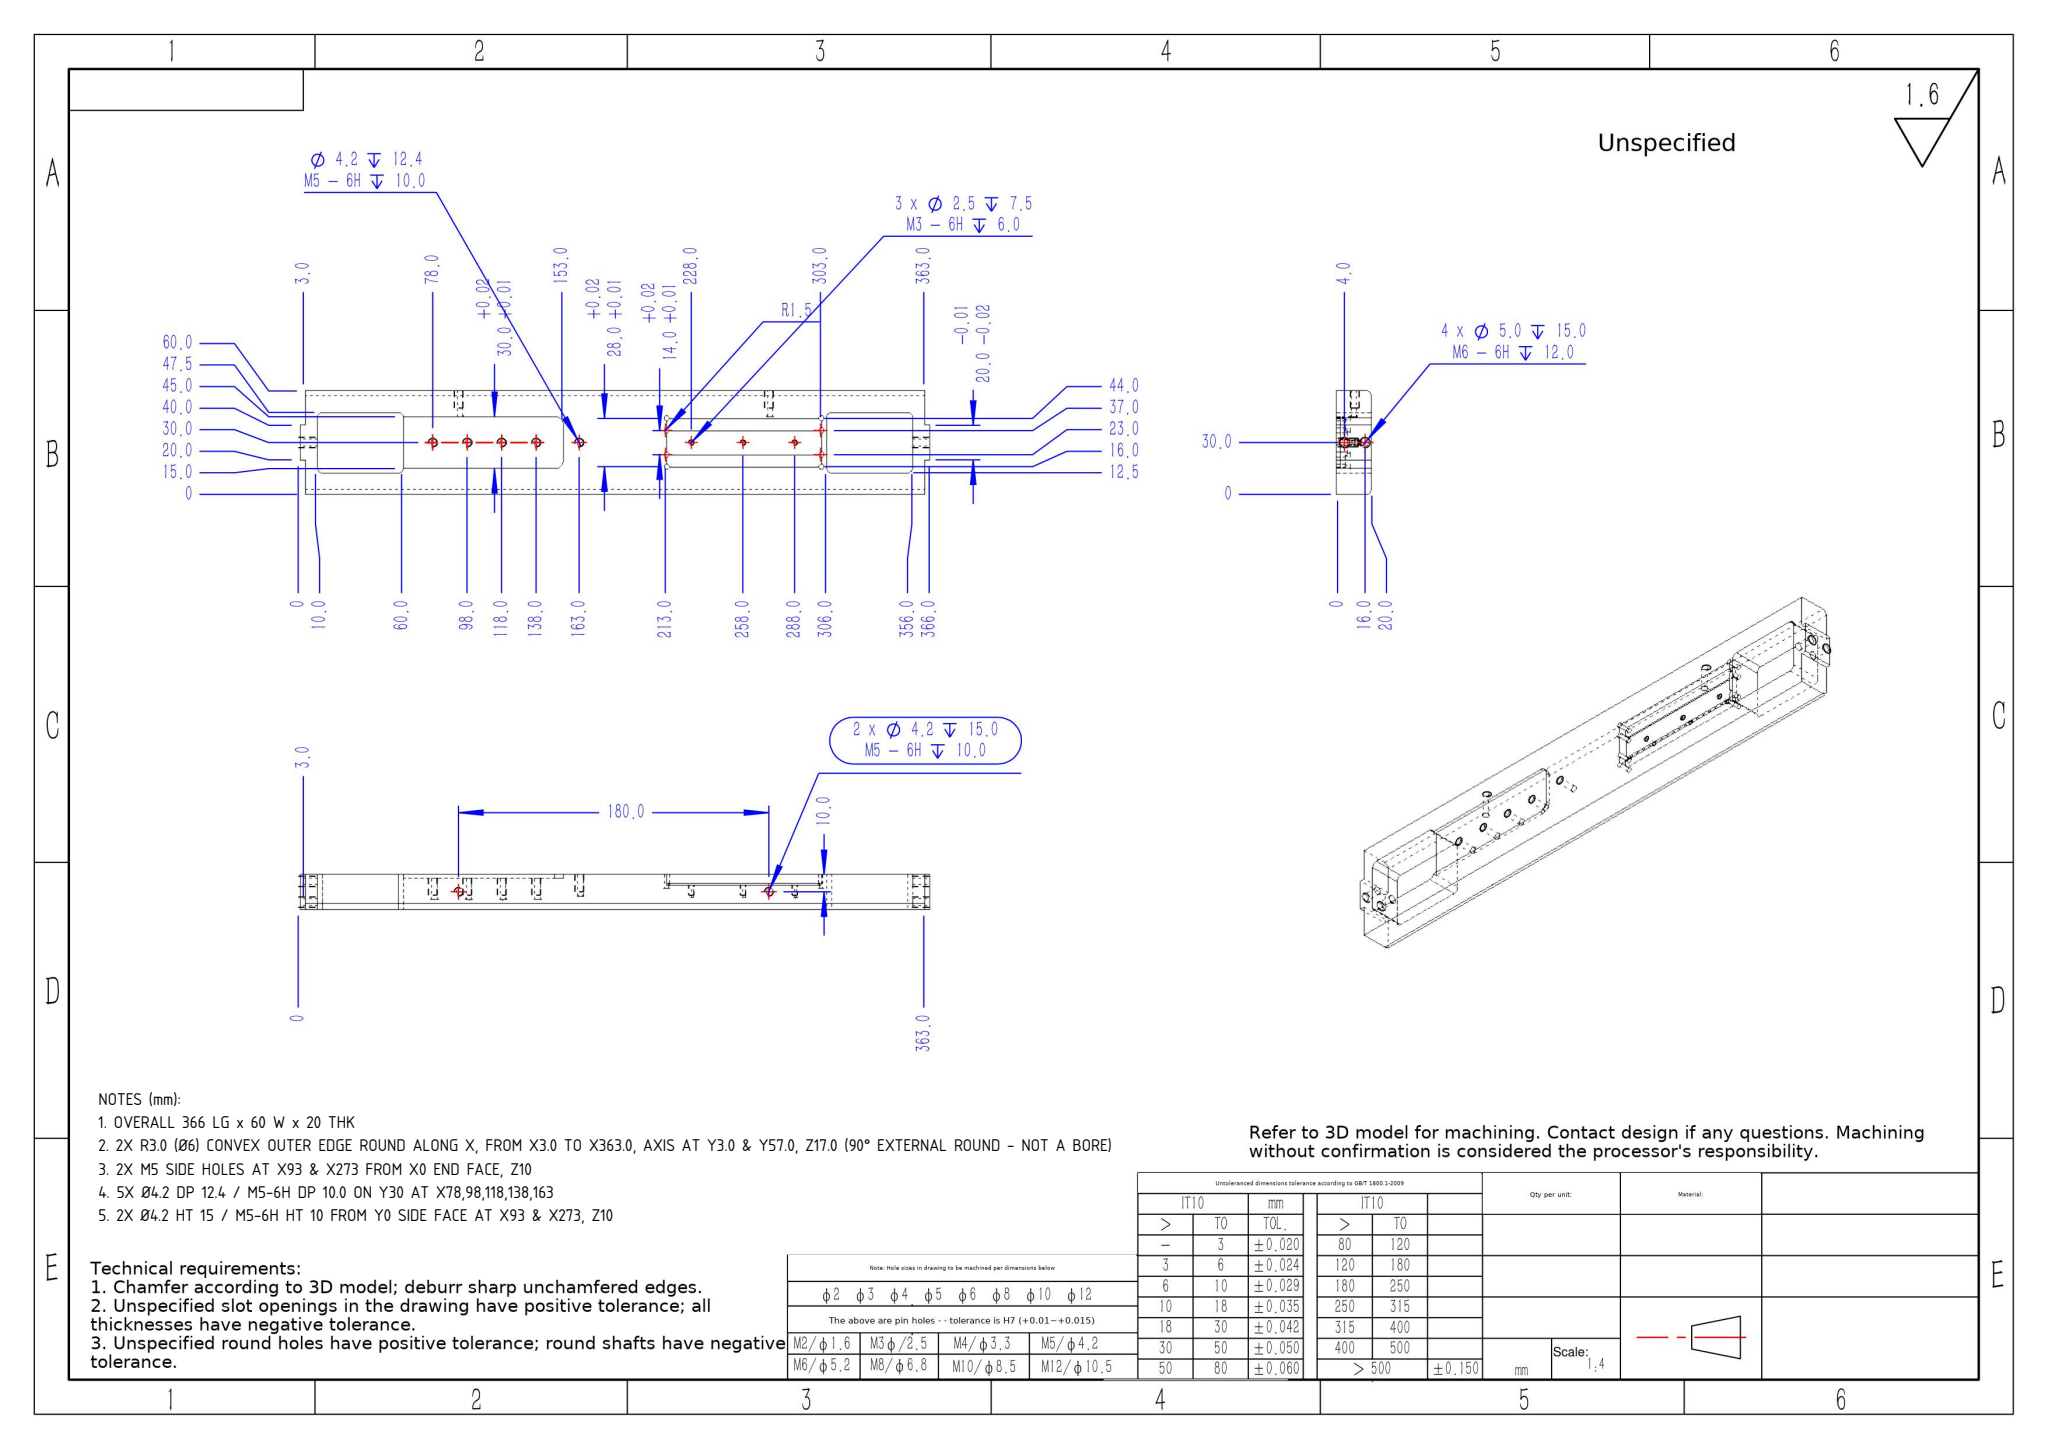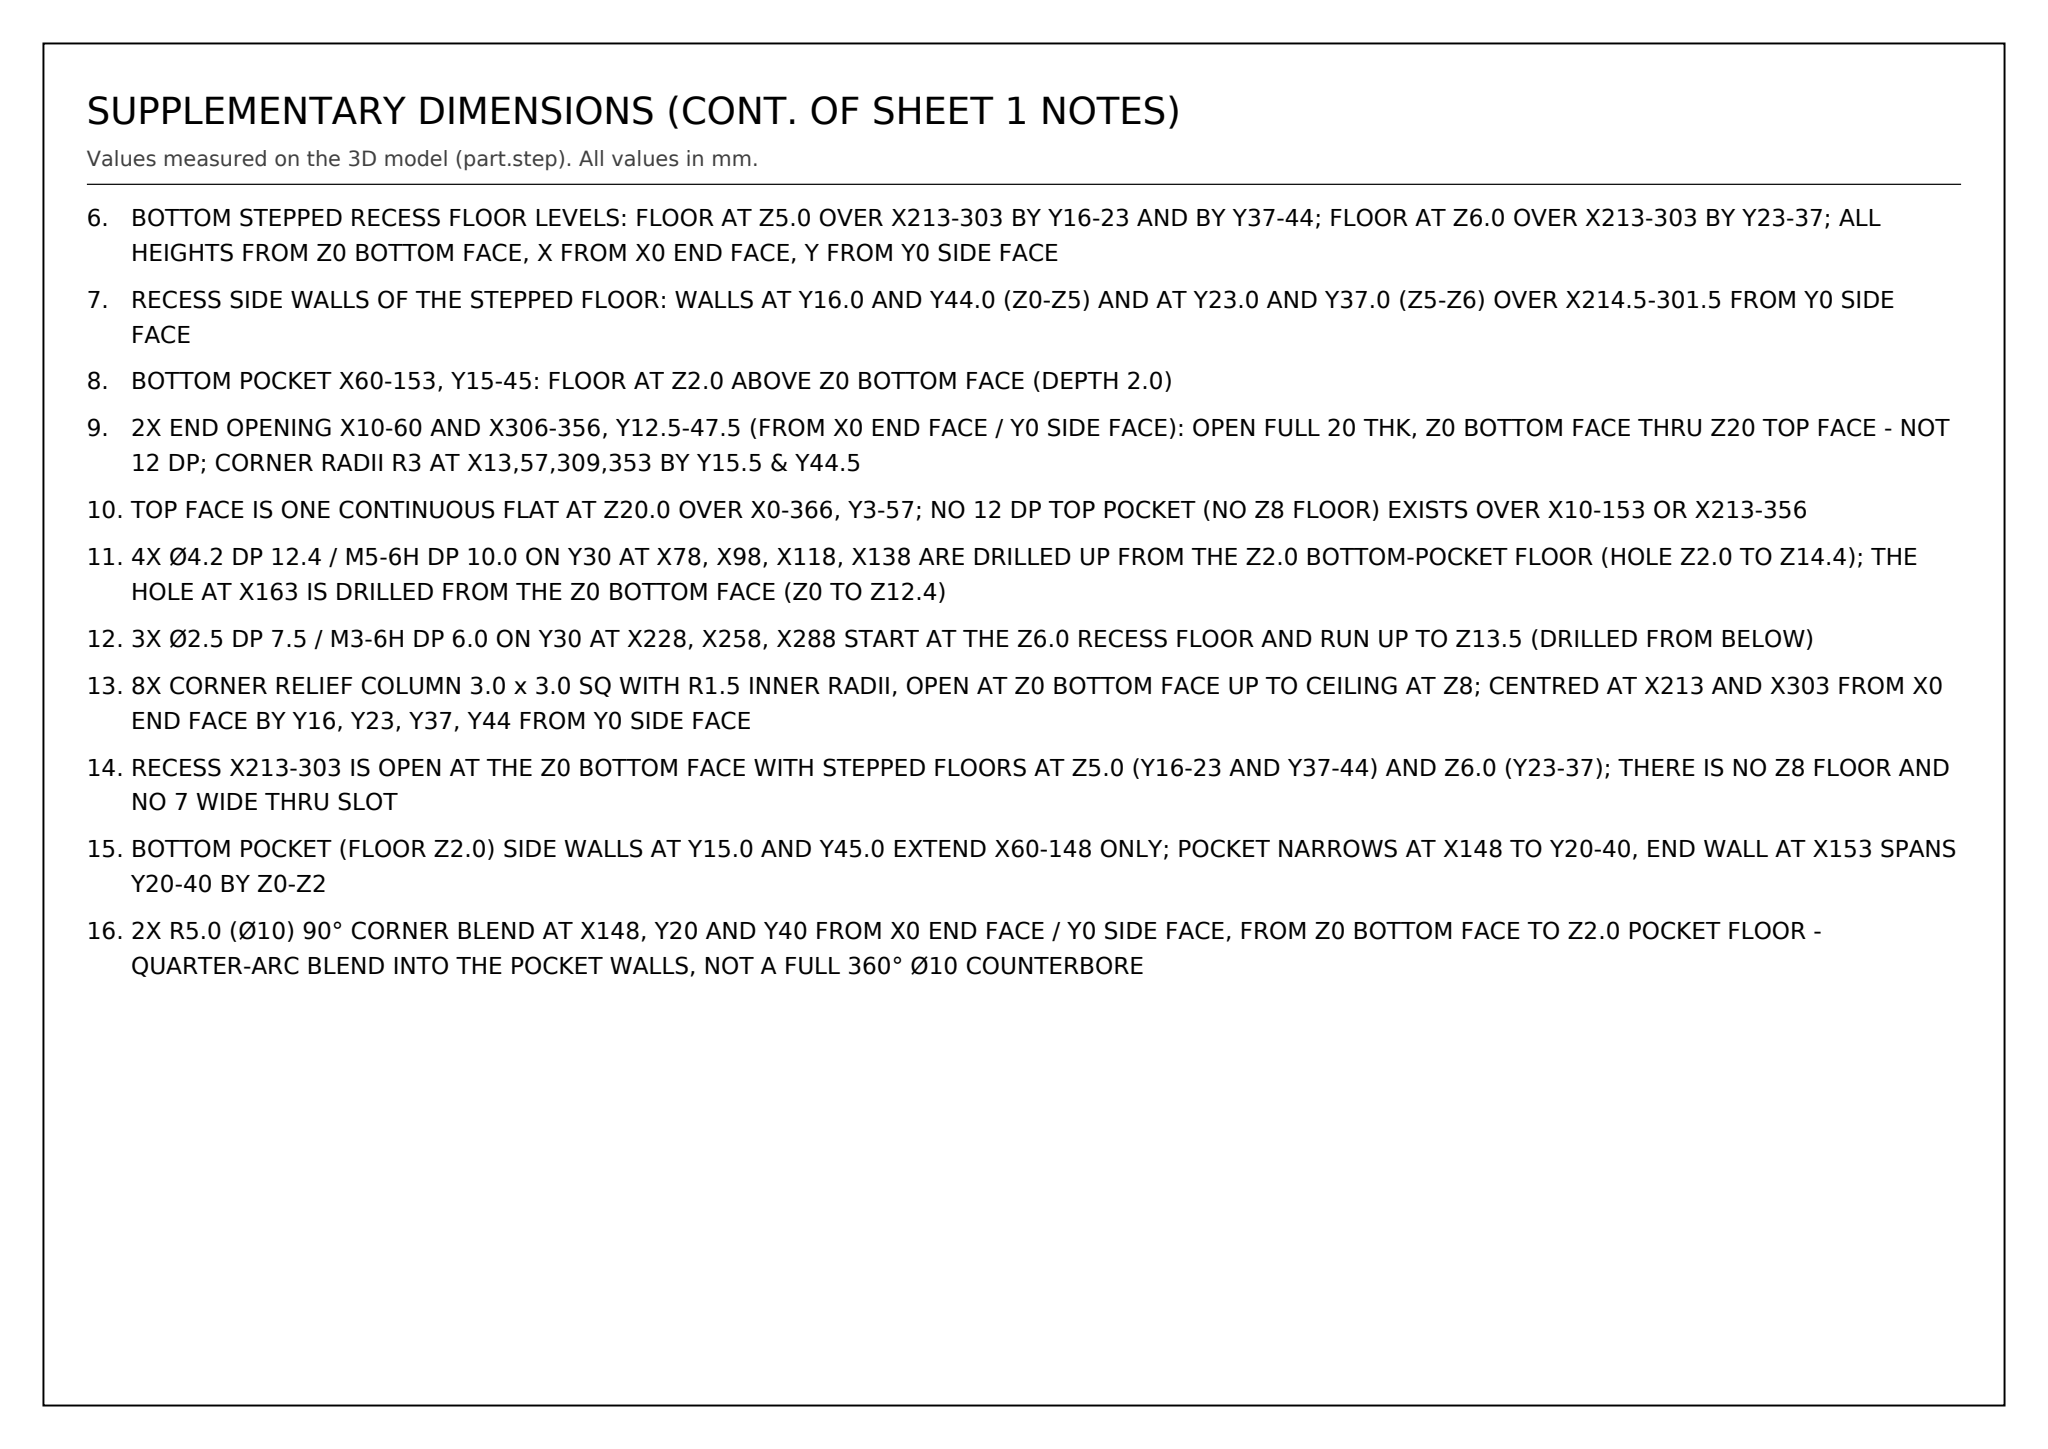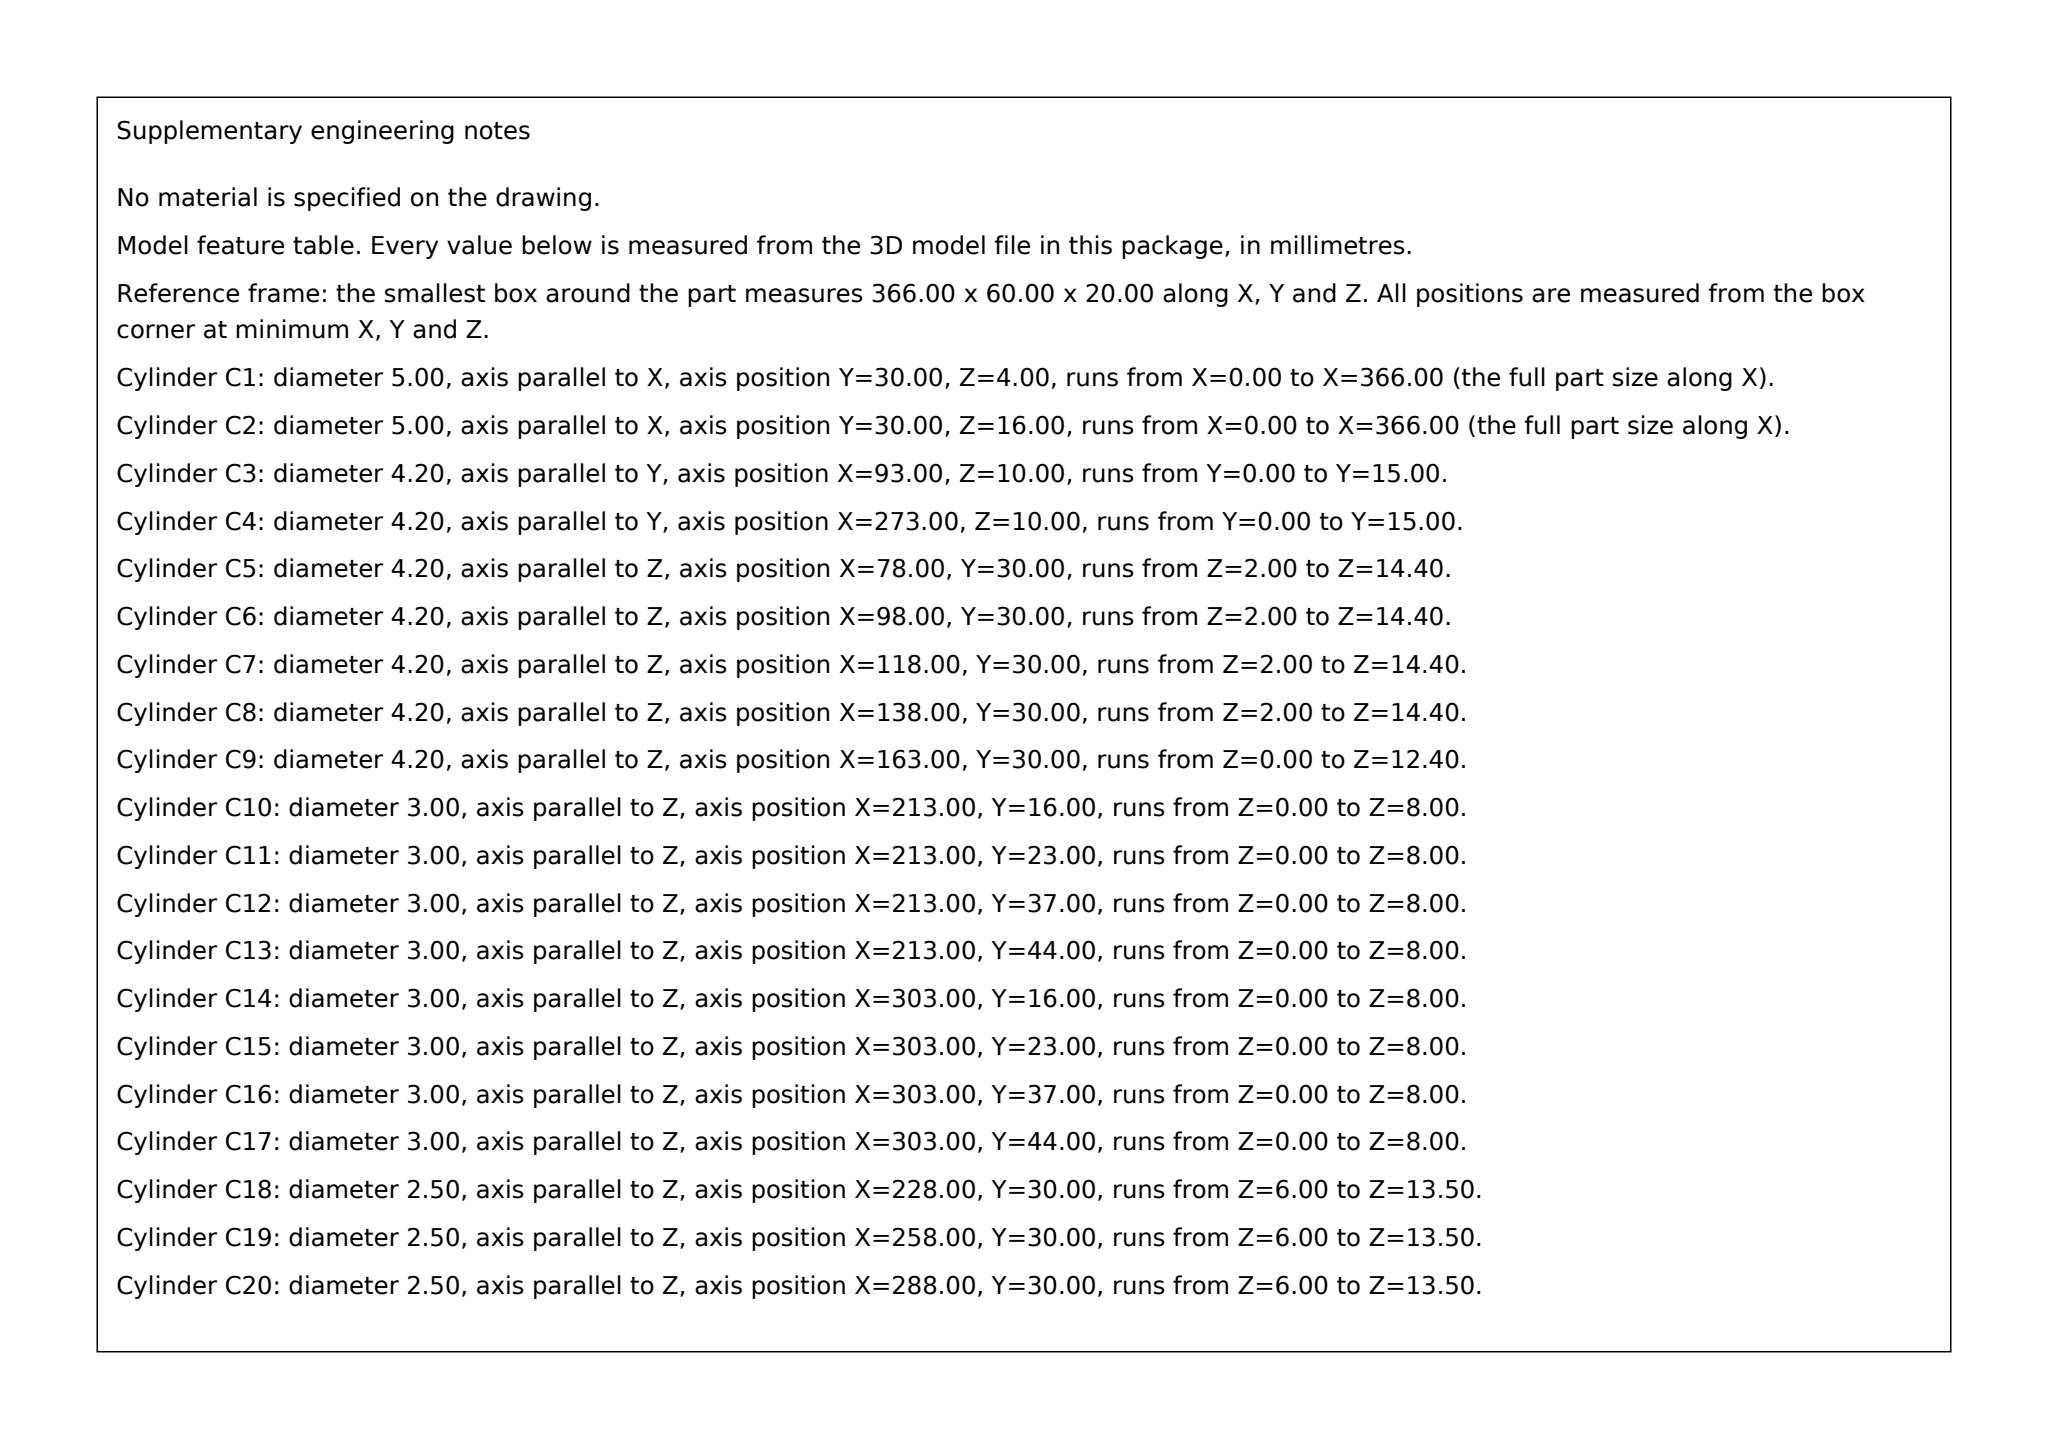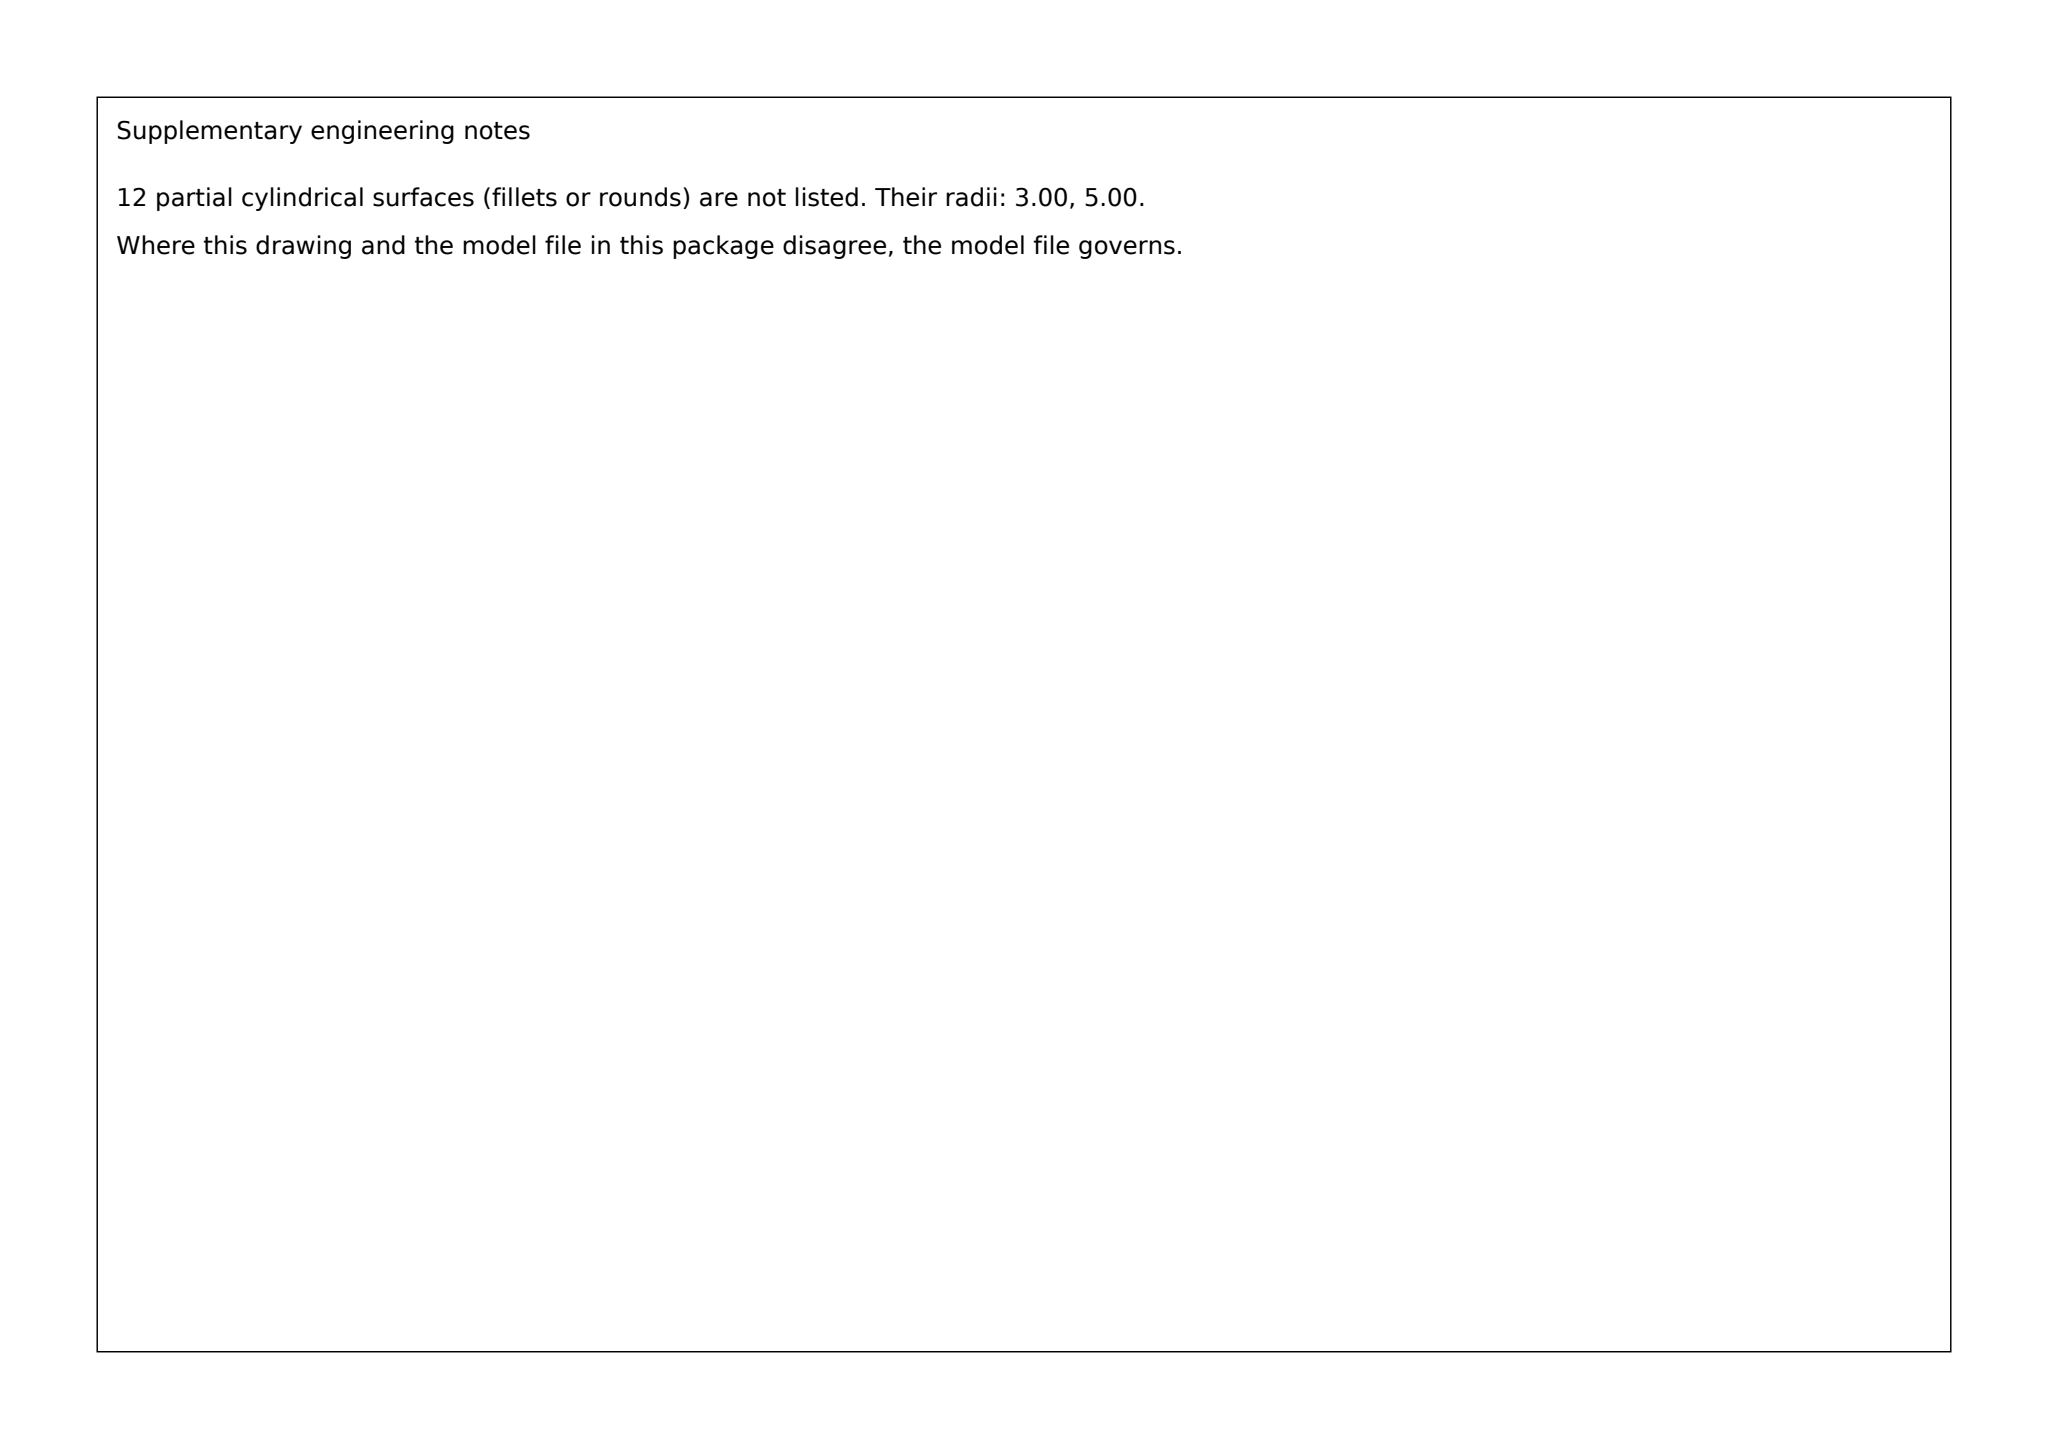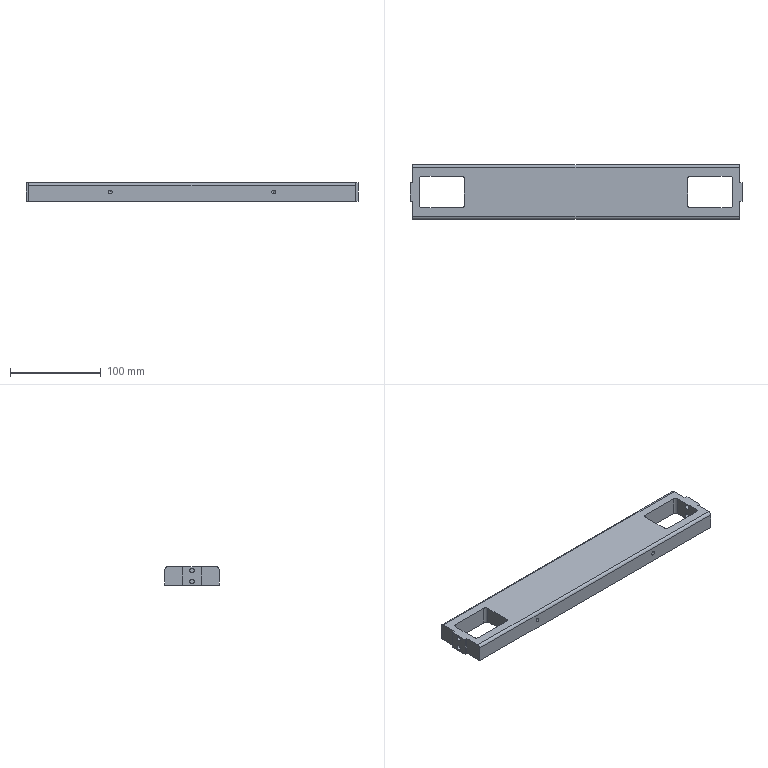Part | SolidWorks | mm | 1 solid | 123 faces | box 366 x 60 x 20 mm | volume 341346 mm3 | cylinder 56 | plane 47 | cone 20 | commonest cylinder face diameters 3 x16 4.2 x14 6 x10 5 x8 2.5 x6 10 x2
Drawing notes:
OVERALL 366 LG x 60 W x 20 THK | from the solid: bbox_xyz = [366.0, 60.0, 20.0]
2X R3.0 (Ø6) CONVEX OUTER EDGE ROUND ALONG X, FROM X3.0 TO X363.0, AXIS AT Y3.0 & Y57.0, Z17.0 (90° EXTERNAL ROUND - NOT A BORE) | from the solid: cylinders: ["convex arc (round/outer radius)", 6.0, "x", [null, 3.0, 17.0], from 3.0 to 363.0, arc_deg 90] and ["convex arc (round/outer radius)", 6.0, "x", [null, 57.0, 17.0], from 3.0 to 363.0, arc_deg 90]; no 360° Ø6 bore along X exists
2X M5 SIDE HOLES AT X93 & X273 FROM X0 END FACE, Z10 | from the solid: Ø4.2 y-axis cyls at [93,-,10] & [273,-,10], L15
5X Ø4.2 DP 12.4 / M5-6H DP 10.0 ON Y30 AT X78,98,118,138,163 | from the solid: Five Ø4.2 z-axis cylinders, 12.4 deep, at y=30.0, x=78/98/118/138/163; 118° ref dia 4.2 drill cones
2X Ø4.2 HT 15 / M5-6H HT 10 FROM Y0 SIDE FACE AT X93 & X273, Z10 | from the solid: cylinders dia 4.2 axis y, pos [93,-,10] and [273,-,10], length 15; bbox Y=0..60, holes normal to Y side face, drilled from the front (Y0) face shown in lower view
BOTTOM STEPPED RECESS FLOOR LEVELS: FLOOR AT Z5.0 OVER X213-303 BY Y16-23 AND BY Y37-44; FLOOR AT Z6.0 OVER X213-303 BY Y23-37; ALL HEIGHTS FROM Z0 BOTTOM FACE, X FROM X0 END FACE, Y FROM Y0 SIDE FACE | from the solid: axis_planes: z=5.0 extent x[213,303] y[16,23] and z=5.0 extent x[213,303] y[37,44]; z=6.0 extent x[213,303] y[23,37]
RECESS SIDE WALLS OF THE STEPPED FLOOR: WALLS AT Y16.0 AND Y44.0 (Z0-Z5) AND AT Y23.0 AND Y37.0 (Z5-Z6) OVER X214.5-301.5 FROM Y0 SIDE FACE | from the solid: axis_planes: y=16.0 and y=44.0 extent x[214.5,301.5] z[0,5]; y=23.0 and y=37.0 extent x[214.5,301.5] z[5,6]
BOTTOM POCKET X60-153, Y15-45: FLOOR AT Z2.0 ABOVE Z0 BOTTOM FACE (DEPTH 2.0) | from the solid: axis_planes: z=2.0 extent x[60,153] y[15,45]; walls y=15.0 and y=45.0 extent x[60,148] z[0,2]; x=60.0 face z[2,20]
2X END OPENING X10-60 AND X306-356, Y12.5-47.5 (FROM X0 END FACE / Y0 SIDE FACE): OPEN FULL 20 THK, Z0 BOTTOM FACE THRU Z20 TOP FACE - NOT 12 DP; CORNER RADII R3 AT X13,57,309,353 BY Y15.5 & Y44.5 | from the solid: axis_planes x=10 and x=356 extent y15.5-44.5 z0-20; x=306 extent y15.5-44.5 z0-20; y=12.5 and y=47.5 extents x13-57 and x309-353, z0-20; cylinders dia 6.0 axis z at (13,15.5),(57,44.5),(309,15.5),(353,44.5) from z0 to z20
TOP FACE IS ONE CONTINUOUS FLAT AT Z20.0 OVER X0-366, Y3-57; NO 12 DP TOP POCKET (NO Z8 FLOOR) EXISTS OVER X10-153 OR X213-356 | from the solid: axis_plane z=20.0 extent x0-366, y3-57 (single face, area 16075); no z-plane at offset 8.0 spanning those X ranges
4X Ø4.2 DP 12.4 / M5-6H DP 10.0 ON Y30 AT X78, X98, X118, X138 ARE DRILLED UP FROM THE Z2.0 BOTTOM-POCKET FLOOR (HOLE Z2.0 TO Z14.4); THE HOLE AT X163 IS DRILLED FROM THE Z0 BOTTOM FACE (Z0 TO Z12.4) | from the solid: cylinders dia 4.2 axis z at (78,30),(98,30),(118,30),(138,30) from 2.0 to 14.4 and at (163,30) from 0.0 to 12.4; axis_plane z=2.0 extent x60-153, y15-45
3X Ø2.5 DP 7.5 / M3-6H DP 6.0 ON Y30 AT X228, X258, X288 START AT THE Z6.0 RECESS FLOOR AND RUN UP TO Z13.5 (DRILLED FROM BELOW) | from the solid: cylinders dia 2.5 axis z at (228,30),(258,30),(288,30) from 6.0 to 13.5; axis_plane z=6.0 extent x213-303, y23-37
8X CORNER RELIEF COLUMN 3.0 x 3.0 SQ WITH R1.5 INNER RADII, OPEN AT Z0 BOTTOM FACE UP TO CEILING AT Z8; CENTRED AT X213 AND X303 FROM X0 END FACE BY Y16, Y23, Y37, Y44 FROM Y0 SIDE FACE | from the solid: z=8.0 planes at x[211.5,214.5] and x[301.5,304.5] by y[14.5,17.5],[21.5,24.5],[35.5,38.5],[42.5,45.5]; Ø3.0 z-arcs (R1.5) at (213/303, 16/23/37/44) from z0 to z8
RECESS X213-303 IS OPEN AT THE Z0 BOTTOM FACE WITH STEPPED FLOORS AT Z5.0 (Y16-23 AND Y37-44) AND Z6.0 (Y23-37); THERE IS NO Z8 FLOOR AND NO 7 WIDE THRU SLOT | from the solid: z=5.0 planes x[213,303] y[16,23] and y[37,44]; z=6.0 plane x[213,303] y[23,37]; no z=8 floor over this area except the 3x3 relief tops
BOTTOM POCKET (FLOOR Z2.0) SIDE WALLS AT Y15.0 AND Y45.0 EXTEND X60-148 ONLY; POCKET NARROWS AT X148 TO Y20-40, END WALL AT X153 SPANS Y20-40 BY Z0-Z2 | from the solid: y=15.0 and y=45.0 planes extent x[60,148] z[0,2]; x=153.0 plane extent y[20,40] z[0,2]; z=2.0 floor x[60,153] y[15,45]
2X R5.0 (Ø10) 90° CORNER BLEND AT X148, Y20 AND Y40 FROM X0 END FACE / Y0 SIDE FACE, FROM Z0 BOTTOM FACE TO Z2.0 POCKET FLOOR - QUARTER-ARC BLEND INTO THE POCKET WALLS, NOT A FULL 360° Ø10 COUNTERBORE | from the solid: concave arcs dia 10.0, z axis, at (148,20) and (148,40), from z0.0 to z2.0, arc_deg 90
build123d program:
from build123d import *

# Parameters (mm, degrees)
SKETCH1_W             = 360
SKETCH1_H             = 60
BOSS_EXTRUDE1_DEPTH   = 10
SKETCH2_W             = 20
SKETCH2_H             = 20
BOSS_EXTRUDE2_DEPTH   = 3
SKETCH5_W             = 90
SKETCH5_H             = 28
CUT_EXTRUDE1_DEPTH    = 5
SKETCH6_W             = 90
SKETCH6_H             = 14
CUT_EXTRUDE2_DEPTH    = 1
SKETCH7_R             = 1.5
CUT_EXTRUDE3_DEPTH    = 8
M3_TAPPED_HOLE2_D     = 2.5
M3_TAPPED_HOLE2_DEPTH = 7.5
M3_TAPPED_HOLE2_TIP   = 0.7511
SKETCH12_W            = 50
SKETCH12_H            = 35
CUT_EXTRUDE4_DEPTH    = 46
FILLET1_R             = 3
FILLET1_OF_MIRROR4_R  = 3
SKETCH13_W            = 106.732
SKETCH13_H            = 30
CUT_EXTRUDE5_DEPTH    = 2
FILLET2_R             = 5
LPATTERN1_COUNT       = 4
LPATTERN1_PITCH       = 20
M5_TAPPED_HOLE2_D     = 4.2
M5_TAPPED_HOLE2_DEPTH = 12.4
M5_TAPPED_HOLE2_TIP   = 1.262
FILLET3_R             = 3
M5_TAPPED_HOLE3_D     = 4.2
M5_TAPPED_HOLE3_DEPTH = 15
M5_TAPPED_HOLE3_TIP   = 1.262


with BuildPart() as part:
    # Sketch1 → Boss-Extrude1 (new, symmetric)
    with BuildSketch(Plane.XY):
        Rectangle(SKETCH1_W, SKETCH1_H)
    extrude(amount=BOSS_EXTRUDE1_DEPTH, both=True)

    # Sketch2 → Boss-Extrude2 (add)
    with BuildSketch(Plane(origin=(180, 0, 0), x_dir=(0, 0, -1), z_dir=(1, 0, 0))):
        Rectangle(SKETCH2_W, SKETCH2_H)
    boss_extrude2 = extrude(amount=BOSS_EXTRUDE2_DEPTH)

    # Mirror1: Boss-Extrude2 across plane
    add(boss_extrude2.mirror(Plane(origin=(0, 0, 0), x_dir=(0, 0, 1), z_dir=(1, 0, 0))))

    # Sketch4 → M6 Tapped Hole1 (revolve, cut)
    with BuildSketch(Plane(origin=(183, 0, 6), x_dir=(0, 0, -1), z_dir=(0, 1, 0))):
        Polygon((0, 0), (0, 16.502), (2.5, 15), (2.5, 0), align=None)
    m6_tapped_hole1 = revolve(axis=Axis((189.35, 0, 6), (-1, 0, 0)), mode=Mode.SUBTRACT)

    # Mirror2: M6 Tapped Hole1 across plane
    add(m6_tapped_hole1.mirror(Plane.XY), mode=Mode.SUBTRACT)

    # Mirror3: M6 Tapped Hole1 across plane
    add(m6_tapped_hole1.mirror(Plane(origin=(0, 0, 0), x_dir=(0, 0, 1), z_dir=(1, 0, 0))), mode=Mode.SUBTRACT)

    # Mirror3 copy 1 sketch → Mirror3 copy 1 (revolve, cut)
    with BuildSketch(Plane(origin=(-183, 0, -6), x_dir=(0, 0, 1), z_dir=(0, 1, 0))):
        Polygon((0, 0), (0, 16.502), (2.5, 15), (2.5, 0), align=None)
    revolve(axis=Axis((-189.35, 0, -6), (1, 0, 0)), mode=Mode.SUBTRACT)

    # Sketch5 → Cut-Extrude1 (cut)
    with BuildSketch(Plane(origin=(0, 0, -10), x_dir=(-1, 0, 0), z_dir=(0, 0, -1))):
        with Locations((-75, 0)):
            Rectangle(SKETCH5_W, SKETCH5_H)
    extrude(amount=-CUT_EXTRUDE1_DEPTH, mode=Mode.SUBTRACT)

    # Sketch6 → Cut-Extrude2 (cut)
    with BuildSketch(Plane(origin=(0, 0, -5), x_dir=(-1, 0, 0), z_dir=(0, 0, -1))):
        with Locations((-75, 0)):
            Rectangle(SKETCH6_W, SKETCH6_H)
    extrude(amount=-CUT_EXTRUDE2_DEPTH, mode=Mode.SUBTRACT)

    # Sketch7 → Cut-Extrude3 (cut)
    with BuildSketch(Plane(origin=(0, 0, -10), x_dir=(-1, 0, 0), z_dir=(0, 0, -1))):
        with Locations((-120, -14)):
            Circle(SKETCH7_R)
        with Locations((-120, -7)):
            Circle(SKETCH7_R)
        with Locations((-120, 7)):
            Circle(SKETCH7_R)
        with Locations((-120, 14)):
            Circle(SKETCH7_R)
        with Locations((-30, 14)):
            Circle(SKETCH7_R)
        with Locations((-30, 7)):
            Circle(SKETCH7_R)
        with Locations((-30, -7)):
            Circle(SKETCH7_R)
        with Locations((-30, -14)):
            Circle(SKETCH7_R)
    extrude(amount=-CUT_EXTRUDE3_DEPTH, mode=Mode.SUBTRACT)

    # M3 Tapped Hole2
    with Locations(Plane(origin=(0, 0, -4), x_dir=(-1, 0, 0), z_dir=(0, 0, -1))):
        with Locations((-105, 0), (-75, 0), (-45, 0)):
            Hole(M3_TAPPED_HOLE2_D / 2, depth=M3_TAPPED_HOLE2_DEPTH)
            with Locations((0, 0, -(M3_TAPPED_HOLE2_DEPTH + M3_TAPPED_HOLE2_TIP / 2))):  # 118° drill point
                Cone(0, M3_TAPPED_HOLE2_D / 2, M3_TAPPED_HOLE2_TIP, mode=Mode.SUBTRACT)

    # Sketch12 → Cut-Extrude4 (cut)
    with BuildSketch(Plane(origin=(0, 0, -10), x_dir=(-1, 0, 0), z_dir=(0, 0, -1))):
        with Locations((-148, 0)):
            Rectangle(SKETCH12_W, SKETCH12_H)
    cut_extrude4 = extrude(amount=-CUT_EXTRUDE4_DEPTH, mode=Mode.SUBTRACT)

    # Fillet1
    fillet1_edges = [part.edges().sort_by_distance(p)[0] for p in [
        (173, 17.5, 0),
        (123, 17.5, 0),
        (123, -17.5, 0),
        (173, -17.5, 0),
    ]]
    fillet(fillet1_edges, radius=FILLET1_R)

    # Mirror4: Cut-Extrude4 across plane
    add(cut_extrude4.mirror(Plane(origin=(0, 0, 0), x_dir=(0, 0, 1), z_dir=(1, 0, 0))), mode=Mode.SUBTRACT)

    # Fillet1 of Mirror4
    fillet1_of_mirror4_edges = [part.edges().sort_by_distance(p)[0] for p in [
        (-173, 17.5, 0),
        (-123, 17.5, 0),
        (-123, -17.5, 0),
        (-173, -17.5, 0),
    ]]
    fillet(fillet1_of_mirror4_edges, radius=FILLET1_OF_MIRROR4_R)

    # Sketch13 → Cut-Extrude5 (cut)
    with BuildSketch(Plane(origin=(0, 0, -10), x_dir=(-1, 0, 0), z_dir=(0, 0, -1))):
        with Locations((83.366, 0)):
            Rectangle(SKETCH13_W, SKETCH13_H)
    extrude(amount=-CUT_EXTRUDE5_DEPTH, mode=Mode.SUBTRACT)

    # Fillet2
    fillet2_edges = [part.edges().sort_by_distance(p)[0] for p in [
        (-30, 15, -9),
        (-30, -15, -9),
    ]]
    fillet(fillet2_edges, radius=FILLET2_R)

    # Sketch15 → M5 Tapped Hole1 (revolve, cut)
    with BuildSketch(Plane(origin=(-45, 0, -8), x_dir=(0, 1, 0), z_dir=(1, 0, 0))):
        Polygon((0, 0), (0, 13.662), (2.1, 12.4), (2.1, 0), align=None)
    m5_tapped_hole1 = revolve(axis=Axis((-45, 0, -14.35), (0, 0, 1)), mode=Mode.SUBTRACT)

    # LPattern1: M5 Tapped Hole1 ×4
    with Locations(*[(-i * LPATTERN1_PITCH, 0, 0) for i in range(1, LPATTERN1_COUNT)]):
        add(m5_tapped_hole1, mode=Mode.SUBTRACT)

    # M5 Tapped Hole2
    with Locations(Plane(origin=(0, 0, -10), x_dir=(-1, 0, 0), z_dir=(0, 0, -1))):
        with Locations((20, 0)):
            Hole(M5_TAPPED_HOLE2_D / 2, depth=M5_TAPPED_HOLE2_DEPTH)
            with Locations((0, 0, -(M5_TAPPED_HOLE2_DEPTH + M5_TAPPED_HOLE2_TIP / 2))):  # 118° drill point
                Cone(0, M5_TAPPED_HOLE2_D / 2, M5_TAPPED_HOLE2_TIP, mode=Mode.SUBTRACT)

    # Fillet3
    fillet3_edges = [part.edges().sort_by_distance(p)[0] for p in [
        (0, -30, 10),
        (0, 30, 10),
    ]]
    fillet(fillet3_edges, radius=FILLET3_R)

    # M5 Tapped Hole3
    with Locations(Plane(origin=(0, -30, 0), x_dir=(-1, 0, 0), z_dir=(0, -1, 0))):
        with Locations((-90, 0), (90, 0)):
            Hole(M5_TAPPED_HOLE3_D / 2, depth=M5_TAPPED_HOLE3_DEPTH)
            with Locations((0, 0, -(M5_TAPPED_HOLE3_DEPTH + M5_TAPPED_HOLE3_TIP / 2))):  # 118° drill point
                Cone(0, M5_TAPPED_HOLE3_D / 2, M5_TAPPED_HOLE3_TIP, mode=Mode.SUBTRACT)


solid = part.part